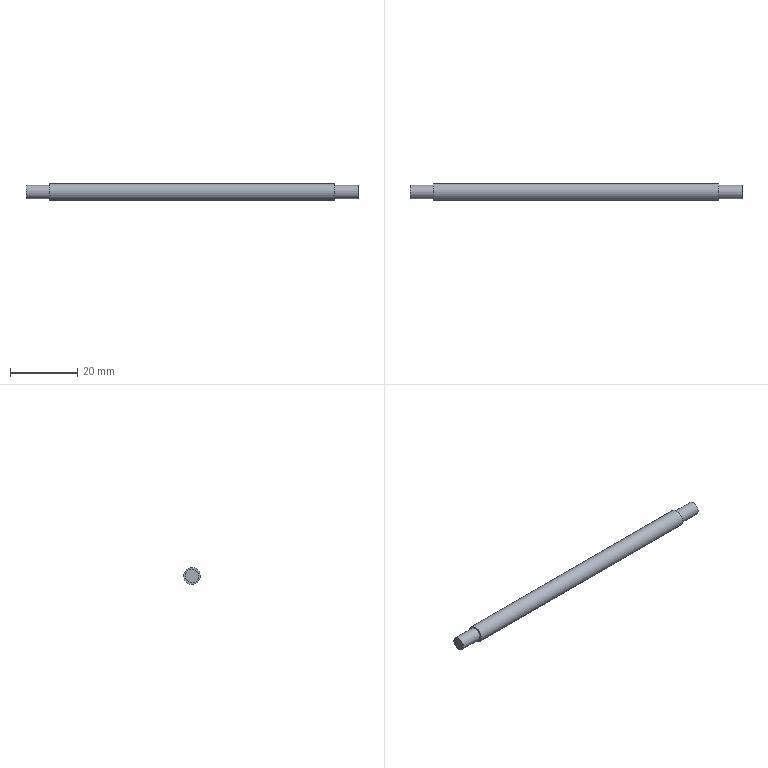Component | NX | LINK_2 | 1 solid | 7 faces | volume 1845 mm3 | plane 4 | cylinder 3 | commonest cylinder face diameters 4 x2 5 x1